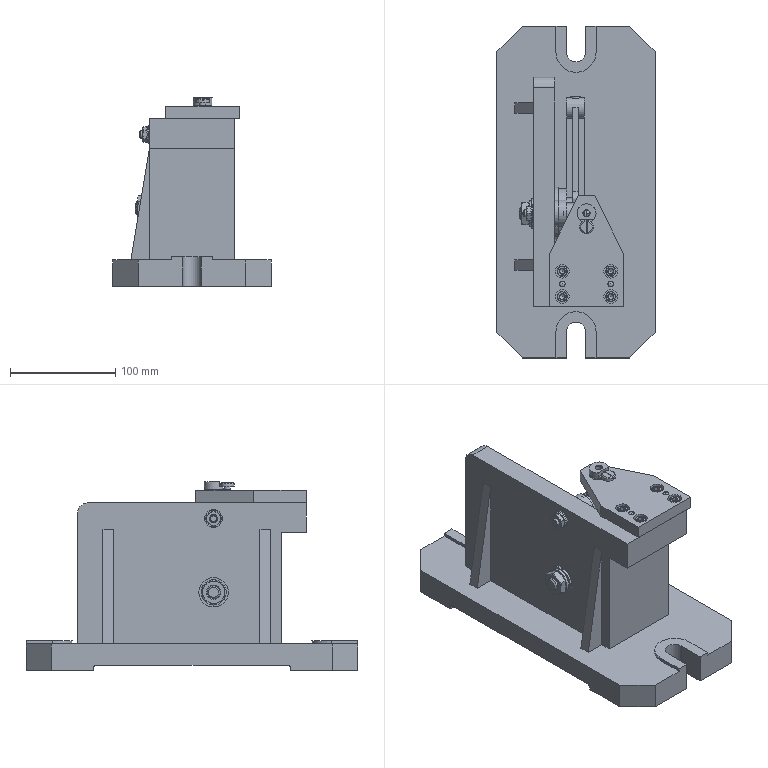Assembly | NX | mm | 33 component files | 33 solids | 690 faces | box 150 x 315 x 179 mm | volume 1859455 mm3 | plane 344 | cone 182 | cylinder 136 | torus 24 | sphere 4 | commonest cylinder face diameters 13 x11 18 x9 7 x8 10 x6 6 x6 5 x6 15 x6 9 x5
Bill of materials:
unnamed part 1 | 1 |  | Flanged cylindrical bushing: a plain cylindrical body with a short, larger-diameter flange at one end and a straight through bore along the axis.
unnamed part 2 | 1 |  | L-shaped lever or bell-crank-like link: two tapered arms meet at a filleted corner. There are three cylindrical bosses, each with a through hole: a large one at the corner and one at each arm end. The arms have recessed webs/channels, and one end boss has a small radial hole or pin feature.
unnamed part 3 | 1 |  | Stepped turned shaft or pin: a long small-diameter end section, a mid-diameter step, a narrow groove, a raised collar, a short tapered transition, a larger cylindrical section and a short small-diameter end, with chamfered ends.
GB-T97_1-2002,M12 | 1 |  | Thin flat annular ring (plain washer-like disc) with a central circular through-hole; flat parallel faces and plain cylindrical outer and inner edges.
GB-T70.1-2000,M3x12 | 4 |  | Hexagon Socket Head Cap Screw, GB-T 70.1-2000,M3x12
unnamed part 4 | 1 |  | Slotted-head pin: a wide cylindrical head with a chamfered top edge and a straight slot across it, a shorter intermediate-diameter neck, a reduced-diameter undercut section, and a cylindrical shank with a chamfered tip.
GB-T41-2000,M6x1 | 1 |  | Hexagonal prism with a central circular through-bore and conical chamfers at both ends (hex-nut-like body); height somewhat greater than the across-flats width.
unnamed part 5 | 1 |  | Plain cylindrical sleeve or spacer tube with a fairly thick wall, a through bore, and small chamfers on the outer and inner edges at both ends.
GB-T6172_1-2000,M8x1.25 | 1 |  | Hexagon Thin Nut, Chamfered, GB-T 6172.1-2000,M8x1.25
unnamed part 6 | 1 |  | Stepped pin: a long chamfered cylindrical shank, a larger-diameter step, a narrow groove, a thin raised collar, a short neck, and an end section with two parallel flats and a chamfered end.
unnamed part 7 | 1 |  | Flat annular ring or flange plate with a large central bore and four small through holes evenly spaced on a bolt circle.
GB-T96_1-2002,M6 | 1 |  | Thin flat annular disc with a relatively small central circular through-hole and a wide flat rim (fender/large-OD washer-like ring).
unnamed part 8 | 1 |  | Flanged cylindrical bushing with a through hole that is chamfered or countersunk at the top. The flange has a partial-depth flat or step cut on one side, and there is a small step between the flange and the cylindrical body.
unnamed part 9 | 1 |  | Thick annular ring with a large central bore and four through holes evenly spaced close to the bore. In the isometric view the holes seem to break into or notch the bore wall.
unnamed part 10 | 1 |  | Flanged cylindrical bushing: a cylindrical body with a thin, larger-diameter flange at one end and a through bore. Proportionally it is similar to unnamed part 1.
unnamed part 11 | 1 |  | Flat plate with a five-sided outline: a rectangle with one end tapered to a narrow flat tip. It has one large through hole near the tip with a small hole below it, and two columns of three holes (large-small-large) along the wide end.
unnamed part 12 | 1 |  | Fixture-like bracket body: a rectangular base plate with chamfered corners and U-shaped slots at both ends, and an upright plate on top with a tapered support on one side and a stepped block at the top. The upright has two hole patterns, each a central hole with four small surrounding holes. Rows of small holes sit on the top block, and the base has small pockets, slots and an underside relief.
unnamed part 13 | 1 |  | Thin flat annular ring (plain washer/ring shape) with a large central bore, narrow radial wall, and what looks like a roughly square rectangular cross-section.
GB-T97_1-2002,M8 | 1 |  | Thin flat annular ring with a central circular through-hole roughly half the outer diameter; plain flat faces and cylindrical edges.
GB-T6172_1-2000,M14x2 | 1 |  | Hexagon Thin Nut, Chamfered, GB-T 6172.1-2000,M14x2
GB-T117_A-2000,5x18 | 2 |  | Solid cylindrical rod/pin with slightly domed (convex) ends at both sides; length roughly three times the diameter; no visible holes, grooves, or steps.
GB-T70.1-2000,M4x12 | 4 |  | Hexagon Socket Head Cap Screw, GB-T 70.1-2000,M4x12
GB-T70.1-2000,M6x20 | 4 |  | Hexagon Socket Head Cap Screw, GB-T 70.1-2000,M6x20
Mates:
1. fix | fixture_body 1 component
2. touch align | drill_template 1 face | fixture_body 1 face
3. touch align | drill_template 1 face | fixture_body 1 face
4. touch align | drill_template 1 face | fixture_body 1 face
5. concentric | locating_bush 1 edge | fixture_body 1 edge
6. concentric | repl_loc_pin 1 edge | locating_bush 1 edge
7. touch align | spacer_sleeve 1 face | fixture_body 1 face
8. touch align | spacer_sleeve 1 face | fixture_body 1 face
9. touch align | spacer_sleeve 1 face | fixture_body 1 face
10. concentric | bushing 1 edge | drill_template 1 edge
11. concentric | repl_drill_bush 1 edge | bushing 1 edge
12. touch align | screw 1 face | drill_template 1 face
13. touch align | screw 1 face | repl_drill_bush 1 face
14. concentric | product 1 edge | spacer_sleeve 1 edge
15. touch align | product 1 face | fixture_body 1 face
16. concentric | washer 1 edge | fixture_body 1 edge
17. concentric | locating_bush_2 1 edge | washer 1 edge
18. concentric | repl_loc_pin_2 1 edge | locating_bush_2 1 edge
19. touch align | spacer_sleeve_2 1 face | fixture_body 1 face
20. concentric | spacer_sleeve_2 1 edge | fixture_body 1 edge
21. concentric | GB-T70_1-2000_M3x12 4 edge | spacer_sleeve_2 1 edge
22. concentric | GB-T70_1-2000_M4x12 4 edge | spacer_sleeve 1 edge
23. bond | spacer_sleeve 1 component | assembly component
24. bond | GB-T70_1-2000_M4x12 4 component | assembly component
25. bond | GB-T70_1-2000_M4x12 3 component | assembly component
26. bond | GB-T70_1-2000_M4x12 2 component | assembly component
27. bond | GB-T70_1-2000_M4x12 1 component | assembly component
28. circular | assembly datumaxis | assembly cartesiancoordinatesystem | assembly cartesiancoordinatesystem | assembly cartesiancoordinatesystem | assembly cartesiancoordinatesystem
29. bond | spacer_sleeve_2 1 component | assembly component
30. bond | GB-T70_1-2000_M3x12 4 component | assembly component
31. bond | GB-T70_1-2000_M3x12 3 component | assembly component
32. bond | GB-T70_1-2000_M3x12 2 component | assembly component
33. bond | GB-T70_1-2000_M3x12 1 component | assembly component
34. circular | assembly datumaxis | assembly cartesiancoordinatesystem | assembly cartesiancoordinatesystem | assembly cartesiancoordinatesystem | assembly cartesiancoordinatesystem
35. concentric | GB-T70_1-2000_M6x20 1 edge | drill_template 1 edge
36. concentric | GB-T70_1-2000_M6x20 4 edge | drill_template 1 edge
37. concentric | GB-T70_1-2000_M6x20 3 edge | drill_template 1 edge
38. concentric | GB-T70_1-2000_M6x20 2 edge | drill_template 1 edge
39. concentric | GB-T97_1-2002_M8 1 edge | fixture_body 1 edge
40. concentric | GB-T97_1-2002_M12 1 edge | fixture_body 1 edge
41. concentric | GB-T6172_1-2000_M8x1_25 1 edge | GB-T97_1-2002_M8 1 edge
42. concentric | GB-T6172_1-2000_M14x2 1 edge | GB-T97_1-2002_M12 1 edge
43. concentric | GB-T96_1-2002_M6 1 edge | product 1 edge
44. concentric | GB-T41-2000_M6x1 1 edge | GB-T96_1-2002_M6 1 edge